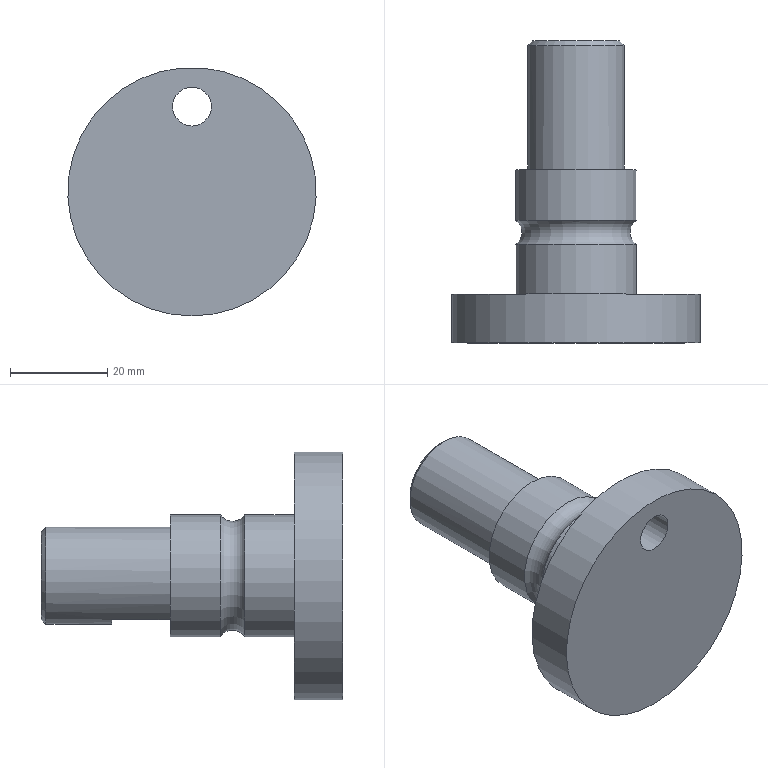Component | NX | 3_CONN_SHAFT | 1 solid | 13 faces | box 51 x 62 x 51 mm | volume 40313 mm3 | plane 6 | cylinder 5 | torus 1 | cone 1 | commonest cylinder face diameters 25 x2 51 x1 8 x1 20 x1
STEP:
#1=CARTESIAN_POINT('',(0.,0.,0.));
#2=DIRECTION('',(0.,0.,1.));
#3=DIRECTION('',(1.,0.,0.));
#4=AXIS2_PLACEMENT_3D('',#1,#2,#3);
#5=CARTESIAN_POINT('',(2.02,26.63,-37.328));
#6=VERTEX_POINT('',#5);
#7=CARTESIAN_POINT('',(2.02,26.63,-24.828));
#8=DIRECTION('',(0.,1.,0.));
#9=DIRECTION('',(0.,0.,-1.));
#10=AXIS2_PLACEMENT_3D('',#7,#8,#9);
#11=CIRCLE('',#10,12.5);
#12=CARTESIAN_POINT('',(2.02,26.63,-24.828));
#13=DIRECTION('',(0.,1.,0.));
#14=DIRECTION('',(0.,0.,-1.));
#15=AXIS2_PLACEMENT_3D('',#12,#13,#14);
#16=CYLINDRICAL_SURFACE('',#15,12.5);
#17=CARTESIAN_POINT('',(0.,0.));
#18=DIRECTION('',(1.,0.));
#19=VECTOR('',#18,1.);
#20=LINE('',#17,#19);
#21=(GEOMETRIC_REPRESENTATION_CONTEXT(2)PARAMETRIC_REPRESENTATION_CONTEXT()REPRESENTATION_CONTEXT('',''));
#22=DEFINITIONAL_REPRESENTATION('',(#20),#21);
#23=PCURVE('',#16,#22);
#24=CARTESIAN_POINT('',(2.02,26.63,-24.828));
#25=DIRECTION('',(0.,1.,0.));
#26=DIRECTION('',(0.,0.,-1.));
#27=AXIS2_PLACEMENT_3D('',#24,#25,#26);
#28=PLANE('',#27);
#29=CARTESIAN_POINT('',(0.,0.));
#30=DIRECTION('',(1.,0.));
#31=AXIS2_PLACEMENT_2D('',#29,#30);
#32=CIRCLE('',#31,12.5);
#33=(GEOMETRIC_REPRESENTATION_CONTEXT(2)PARAMETRIC_REPRESENTATION_CONTEXT()REPRESENTATION_CONTEXT('',''));
#34=DEFINITIONAL_REPRESENTATION('',(#32),#33);
#35=PCURVE('',#28,#34);
#36=SURFACE_CURVE('',#11,(#23,#35),.PCURVE_S1.);
#37=EDGE_CURVE('',#6,#6,#36,.T.);
#38=ORIENTED_EDGE('',*,*,#37,.T.);
#39=CARTESIAN_POINT('',(2.02,36.83,-37.328));
#40=VERTEX_POINT('',#39);
#41=CARTESIAN_POINT('',(2.02,26.63,-37.328));
#42=CARTESIAN_POINT('',(2.02,36.83,-37.328));
#43=B_SPLINE_CURVE_WITH_KNOTS('',1,(#41,#42),.UNSPECIFIED.,.F.,.F.,(2,2),(0.,10.2),.PIECEWISE_BEZIER_KNOTS.);
#44=CARTESIAN_POINT('',(6.283,0.));
#45=DIRECTION('',(0.,1.));
#46=VECTOR('',#45,1.);
#47=LINE('',#44,#46);
#48=(GEOMETRIC_REPRESENTATION_CONTEXT(2)PARAMETRIC_REPRESENTATION_CONTEXT()REPRESENTATION_CONTEXT('',''));
#49=DEFINITIONAL_REPRESENTATION('',(#47),#48);
#50=PCURVE('',#16,#49);
#51=CARTESIAN_POINT('',(0.,0.));
#52=DIRECTION('',(0.,1.));
#53=VECTOR('',#52,1.);
#54=LINE('',#51,#53);
#55=(GEOMETRIC_REPRESENTATION_CONTEXT(2)PARAMETRIC_REPRESENTATION_CONTEXT()REPRESENTATION_CONTEXT('',''));
#56=DEFINITIONAL_REPRESENTATION('',(#54),#55);
#57=PCURVE('',#16,#56);
#58=SEAM_CURVE('',#43,(#50,#57),.PCURVE_S1.);
#59=EDGE_CURVE('',#6,#40,#58,.T.);
#60=ORIENTED_EDGE('',*,*,#59,.T.);
#61=CARTESIAN_POINT('',(2.02,36.83,-12.328));
#62=VERTEX_POINT('',#61);
#63=CARTESIAN_POINT('',(2.02,36.83,-24.828));
#64=DIRECTION('',(0.,-1.,0.));
#65=DIRECTION('',(0.,0.,1.));
#66=AXIS2_PLACEMENT_3D('',#63,#64,#65);
#67=CIRCLE('',#66,12.5);
#68=CARTESIAN_POINT('',(9.425,10.2));
#69=DIRECTION('',(-1.,0.));
#70=VECTOR('',#69,1.);
#71=LINE('',#68,#70);
#72=(GEOMETRIC_REPRESENTATION_CONTEXT(2)PARAMETRIC_REPRESENTATION_CONTEXT()REPRESENTATION_CONTEXT('',''));
#73=DEFINITIONAL_REPRESENTATION('',(#71),#72);
#74=PCURVE('',#16,#73);
#75=CARTESIAN_POINT('',(2.02,39.33,-24.828));
#76=DIRECTION('',(0.,-1.,0.));
#77=DIRECTION('',(0.,0.,1.));
#78=AXIS2_PLACEMENT_3D('',#75,#76,#77);
#79=TOROIDAL_SURFACE('',#78,14.158,3.);
#80=CARTESIAN_POINT('',(0.,2.156));
#81=DIRECTION('',(1.,0.));
#82=VECTOR('',#81,1.);
#83=LINE('',#80,#82);
#84=(GEOMETRIC_REPRESENTATION_CONTEXT(2)PARAMETRIC_REPRESENTATION_CONTEXT()REPRESENTATION_CONTEXT('',''));
#85=DEFINITIONAL_REPRESENTATION('',(#83),#84);
#86=PCURVE('',#79,#85);
#87=SURFACE_CURVE('',#67,(#74,#86),.PCURVE_S1.);
#88=EDGE_CURVE('',#40,#62,#87,.T.);
#89=ORIENTED_EDGE('',*,*,#88,.T.);
#90=CARTESIAN_POINT('',(2.02,36.83,-24.828));
#91=DIRECTION('',(0.,-1.,0.));
#92=DIRECTION('',(0.,0.,1.));
#93=AXIS2_PLACEMENT_3D('',#90,#91,#92);
#94=CIRCLE('',#93,12.5);
#95=CARTESIAN_POINT('',(3.142,10.2));
#96=DIRECTION('',(-1.,0.));
#97=VECTOR('',#96,1.);
#98=LINE('',#95,#97);
#99=(GEOMETRIC_REPRESENTATION_CONTEXT(2)PARAMETRIC_REPRESENTATION_CONTEXT()REPRESENTATION_CONTEXT('',''));
#100=DEFINITIONAL_REPRESENTATION('',(#98),#99);
#101=PCURVE('',#16,#100);
#102=CARTESIAN_POINT('',(0.,2.156));
#103=DIRECTION('',(1.,-0.));
#104=VECTOR('',#103,1.);
#105=LINE('',#102,#104);
#106=(GEOMETRIC_REPRESENTATION_CONTEXT(2)PARAMETRIC_REPRESENTATION_CONTEXT()REPRESENTATION_CONTEXT('',''));
#107=DEFINITIONAL_REPRESENTATION('',(#105),#106);
#108=PCURVE('',#79,#107);
#109=SURFACE_CURVE('',#94,(#101,#108),.PCURVE_S1.);
#110=EDGE_CURVE('',#62,#40,#109,.T.);
#111=ORIENTED_EDGE('',*,*,#110,.T.);
#112=ORIENTED_EDGE('',*,*,#59,.F.);
#113=EDGE_LOOP('',(#38,#60,#89,#111,#112));
#114=FACE_BOUND('',#113,.T.);
#115=ADVANCED_FACE('',(#114),#16,.T.);
#116=CARTESIAN_POINT('',(2.02,26.63,-11.328));
#117=VERTEX_POINT('',#116);
#118=CARTESIAN_POINT('',(2.02,26.63,-7.328));
#119=DIRECTION('',(0.,1.,0.));
#120=DIRECTION('',(0.,0.,-1.));
#121=AXIS2_PLACEMENT_3D('',#118,#119,#120);
#122=CIRCLE('',#121,4.);
#123=CARTESIAN_POINT('',(-17.5,0.));
#124=DIRECTION('',(1.,0.));
#125=AXIS2_PLACEMENT_2D('',#123,#124);
#126=CIRCLE('',#125,4.);
#127=(GEOMETRIC_REPRESENTATION_CONTEXT(2)PARAMETRIC_REPRESENTATION_CONTEXT()REPRESENTATION_CONTEXT('',''));
#128=DEFINITIONAL_REPRESENTATION('',(#126),#127);
#129=PCURVE('',#28,#128);
#130=CARTESIAN_POINT('',(2.02,33.63,-7.328));
#131=DIRECTION('',(0.,-1.,0.));
#132=DIRECTION('',(0.,0.,1.));
#133=AXIS2_PLACEMENT_3D('',#130,#131,#132);
#134=CYLINDRICAL_SURFACE('',#133,4.);
#135=CARTESIAN_POINT('',(9.425,7.));
#136=DIRECTION('',(-1.,0.));
#137=VECTOR('',#136,1.);
#138=LINE('',#135,#137);
#139=(GEOMETRIC_REPRESENTATION_CONTEXT(2)PARAMETRIC_REPRESENTATION_CONTEXT()REPRESENTATION_CONTEXT('',''));
#140=DEFINITIONAL_REPRESENTATION('',(#138),#139);
#141=PCURVE('',#134,#140);
#142=SURFACE_CURVE('',#122,(#129,#141),.PCURVE_S1.);
#143=EDGE_CURVE('',#117,#117,#142,.T.);
#144=ORIENTED_EDGE('',*,*,#143,.F.);
#145=EDGE_LOOP('',(#144));
#146=FACE_BOUND('',#145,.T.);
#147=ORIENTED_EDGE('',*,*,#37,.F.);
#148=EDGE_LOOP('',(#147));
#149=FACE_BOUND('',#148,.T.);
#150=CARTESIAN_POINT('',(2.02,26.63,-50.328));
#151=VERTEX_POINT('',#150);
#152=CARTESIAN_POINT('',(2.02,26.63,-24.828));
#153=DIRECTION('',(0.,-1.,0.));
#154=DIRECTION('',(0.,0.,-1.));
#155=AXIS2_PLACEMENT_3D('',#152,#153,#154);
#156=CIRCLE('',#155,25.5);
#157=CARTESIAN_POINT('',(25.5,0.));
#158=CARTESIAN_POINT('',(25.5,-44.167));
#159=CARTESIAN_POINT('',(-12.75,-22.084));
#160=CARTESIAN_POINT('',(-51.,-0.));
#161=CARTESIAN_POINT('',(-12.75,22.084));
#162=CARTESIAN_POINT('',(25.5,44.167));
#163=CARTESIAN_POINT('',(25.5,0.));
#164=(BOUNDED_CURVE()B_SPLINE_CURVE(2,(#157,#158,#159,#160,#161,#162,#163),.UNSPECIFIED.,.T.,.F.)B_SPLINE_CURVE_WITH_KNOTS((1,2,2,2,2,1),(-2.094,0.,2.094,4.189,6.283,8.378),.UNSPECIFIED.)CURVE()GEOMETRIC_REPRESENTATION_ITEM()RATIONAL_B_SPLINE_CURVE((1.,0.5,1.,0.5,1.,0.5,1.))REPRESENTATION_ITEM(''));
#165=(GEOMETRIC_REPRESENTATION_CONTEXT(2)PARAMETRIC_REPRESENTATION_CONTEXT()REPRESENTATION_CONTEXT('',''));
#166=DEFINITIONAL_REPRESENTATION('',(#164),#165);
#167=PCURVE('',#28,#166);
#168=CARTESIAN_POINT('',(2.02,16.63,-24.828));
#169=DIRECTION('',(0.,1.,0.));
#170=DIRECTION('',(0.,0.,-1.));
#171=AXIS2_PLACEMENT_3D('',#168,#169,#170);
#172=CYLINDRICAL_SURFACE('',#171,25.5);
#173=CARTESIAN_POINT('',(6.283,10.));
#174=DIRECTION('',(-1.,0.));
#175=VECTOR('',#174,1.);
#176=LINE('',#173,#175);
#177=(GEOMETRIC_REPRESENTATION_CONTEXT(2)PARAMETRIC_REPRESENTATION_CONTEXT()REPRESENTATION_CONTEXT('',''));
#178=DEFINITIONAL_REPRESENTATION('',(#176),#177);
#179=PCURVE('',#172,#178);
#180=SURFACE_CURVE('',#156,(#167,#179),.PCURVE_S1.);
#181=EDGE_CURVE('',#151,#151,#180,.T.);
#182=ORIENTED_EDGE('',*,*,#181,.F.);
#183=EDGE_LOOP('',(#182));
#184=FACE_BOUND('',#183,.T.);
#185=ADVANCED_FACE('',(#146,#149,#184),#28,.T.);
#186=CARTESIAN_POINT('',(2.02,16.63,-11.328));
#187=VERTEX_POINT('',#186);
#188=CARTESIAN_POINT('',(2.02,16.63,-7.328));
#189=DIRECTION('',(0.,-1.,0.));
#190=DIRECTION('',(-0.,0.,-1.));
#191=AXIS2_PLACEMENT_3D('',#188,#189,#190);
#192=CIRCLE('',#191,4.);
#193=CARTESIAN_POINT('',(2.02,16.63,-24.828));
#194=DIRECTION('',(0.,-1.,0.));
#195=DIRECTION('',(0.,0.,1.));
#196=AXIS2_PLACEMENT_3D('',#193,#194,#195);
#197=PLANE('',#196);
#198=CARTESIAN_POINT('',(17.5,0.));
#199=DIRECTION('',(-1.,0.));
#200=AXIS2_PLACEMENT_2D('',#198,#199);
#201=CIRCLE('',#200,4.);
#202=(GEOMETRIC_REPRESENTATION_CONTEXT(2)PARAMETRIC_REPRESENTATION_CONTEXT()REPRESENTATION_CONTEXT('',''));
#203=DEFINITIONAL_REPRESENTATION('',(#201),#202);
#204=PCURVE('',#197,#203);
#205=CARTESIAN_POINT('',(3.142,17.));
#206=DIRECTION('',(1.,0.));
#207=VECTOR('',#206,1.);
#208=LINE('',#205,#207);
#209=(GEOMETRIC_REPRESENTATION_CONTEXT(2)PARAMETRIC_REPRESENTATION_CONTEXT()REPRESENTATION_CONTEXT('',''));
#210=DEFINITIONAL_REPRESENTATION('',(#208),#209);
#211=PCURVE('',#134,#210);
#212=SURFACE_CURVE('',#192,(#204,#211),.PCURVE_S1.);
#213=EDGE_CURVE('',#187,#187,#212,.T.);
#214=ORIENTED_EDGE('',*,*,#213,.F.);
#215=EDGE_LOOP('',(#214));
#216=FACE_BOUND('',#215,.T.);
#217=CARTESIAN_POINT('',(2.02,16.63,-50.328));
#218=VERTEX_POINT('',#217);
#219=CARTESIAN_POINT('',(2.02,16.63,-24.828));
#220=DIRECTION('',(0.,1.,0.));
#221=DIRECTION('',(0.,0.,-1.));
#222=AXIS2_PLACEMENT_3D('',#219,#220,#221);
#223=CIRCLE('',#222,25.5);
#224=CARTESIAN_POINT('',(-25.5,0.));
#225=CARTESIAN_POINT('',(-25.5,44.167));
#226=CARTESIAN_POINT('',(12.75,22.084));
#227=CARTESIAN_POINT('',(51.,0.));
#228=CARTESIAN_POINT('',(12.75,-22.084));
#229=CARTESIAN_POINT('',(-25.5,-44.167));
#230=CARTESIAN_POINT('',(-25.5,0.));
#231=(BOUNDED_CURVE()B_SPLINE_CURVE(2,(#224,#225,#226,#227,#228,#229,#230),.UNSPECIFIED.,.T.,.F.)B_SPLINE_CURVE_WITH_KNOTS((1,2,2,2,2,1),(-2.094,0.,2.094,4.189,6.283,8.378),.UNSPECIFIED.)CURVE()GEOMETRIC_REPRESENTATION_ITEM()RATIONAL_B_SPLINE_CURVE((1.,0.5,1.,0.5,1.,0.5,1.))REPRESENTATION_ITEM(''));
#232=(GEOMETRIC_REPRESENTATION_CONTEXT(2)PARAMETRIC_REPRESENTATION_CONTEXT()REPRESENTATION_CONTEXT('',''));
#233=DEFINITIONAL_REPRESENTATION('',(#231),#232);
#234=PCURVE('',#197,#233);
#235=CARTESIAN_POINT('',(0.,0.));
#236=DIRECTION('',(1.,0.));
#237=VECTOR('',#236,1.);
#238=LINE('',#235,#237);
#239=(GEOMETRIC_REPRESENTATION_CONTEXT(2)PARAMETRIC_REPRESENTATION_CONTEXT()REPRESENTATION_CONTEXT('',''));
#240=DEFINITIONAL_REPRESENTATION('',(#238),#239);
#241=PCURVE('',#172,#240);
#242=SURFACE_CURVE('',#223,(#234,#241),.PCURVE_S1.);
#243=EDGE_CURVE('',#218,#218,#242,.T.);
#244=ORIENTED_EDGE('',*,*,#243,.F.);
#245=EDGE_LOOP('',(#244));
#246=FACE_BOUND('',#245,.T.);
#247=ADVANCED_FACE('',(#216,#246),#197,.T.);
#248=ORIENTED_EDGE('',*,*,#181,.T.);
#249=CARTESIAN_POINT('',(2.02,16.63,-50.328));
#250=CARTESIAN_POINT('',(2.02,26.63,-50.328));
#251=B_SPLINE_CURVE_WITH_KNOTS('',1,(#249,#250),.UNSPECIFIED.,.F.,.F.,(2,2),(0.,10.),.PIECEWISE_BEZIER_KNOTS.);
#252=CARTESIAN_POINT('',(0.,0.));
#253=DIRECTION('',(0.,1.));
#254=VECTOR('',#253,1.);
#255=LINE('',#252,#254);
#256=(GEOMETRIC_REPRESENTATION_CONTEXT(2)PARAMETRIC_REPRESENTATION_CONTEXT()REPRESENTATION_CONTEXT('',''));
#257=DEFINITIONAL_REPRESENTATION('',(#255),#256);
#258=PCURVE('',#172,#257);
#259=CARTESIAN_POINT('',(6.283,0.));
#260=DIRECTION('',(0.,1.));
#261=VECTOR('',#260,1.);
#262=LINE('',#259,#261);
#263=(GEOMETRIC_REPRESENTATION_CONTEXT(2)PARAMETRIC_REPRESENTATION_CONTEXT()REPRESENTATION_CONTEXT('',''));
#264=DEFINITIONAL_REPRESENTATION('',(#262),#263);
#265=PCURVE('',#172,#264);
#266=SEAM_CURVE('',#251,(#258,#265),.PCURVE_S1.);
#267=EDGE_CURVE('',#218,#151,#266,.T.);
#268=ORIENTED_EDGE('',*,*,#267,.F.);
#269=ORIENTED_EDGE('',*,*,#243,.T.);
#270=ORIENTED_EDGE('',*,*,#267,.T.);
#271=EDGE_LOOP('',(#248,#268,#269,#270));
#272=FACE_BOUND('',#271,.T.);
#273=ADVANCED_FACE('',(#272),#172,.T.);
#274=ORIENTED_EDGE('',*,*,#143,.F.);
#275=CARTESIAN_POINT('',(2.02,26.63,-11.328));
#276=CARTESIAN_POINT('',(2.02,16.63,-11.328));
#277=B_SPLINE_CURVE_WITH_KNOTS('',1,(#275,#276),.UNSPECIFIED.,.F.,.F.,(2,2),(7.,17.),.PIECEWISE_BEZIER_KNOTS.);
#278=CARTESIAN_POINT('',(9.425,0.));
#279=DIRECTION('',(0.,1.));
#280=VECTOR('',#279,1.);
#281=LINE('',#278,#280);
#282=(GEOMETRIC_REPRESENTATION_CONTEXT(2)PARAMETRIC_REPRESENTATION_CONTEXT()REPRESENTATION_CONTEXT('',''));
#283=DEFINITIONAL_REPRESENTATION('',(#281),#282);
#284=PCURVE('',#134,#283);
#285=CARTESIAN_POINT('',(3.142,0.));
#286=DIRECTION('',(0.,1.));
#287=VECTOR('',#286,1.);
#288=LINE('',#285,#287);
#289=(GEOMETRIC_REPRESENTATION_CONTEXT(2)PARAMETRIC_REPRESENTATION_CONTEXT()REPRESENTATION_CONTEXT('',''));
#290=DEFINITIONAL_REPRESENTATION('',(#288),#289);
#291=PCURVE('',#134,#290);
#292=SEAM_CURVE('',#277,(#284,#291),.PCURVE_S1.);
#293=EDGE_CURVE('',#117,#187,#292,.T.);
#294=ORIENTED_EDGE('',*,*,#293,.T.);
#295=ORIENTED_EDGE('',*,*,#213,.F.);
#296=ORIENTED_EDGE('',*,*,#293,.F.);
#297=EDGE_LOOP('',(#274,#294,#295,#296));
#298=FACE_BOUND('',#297,.F.);
#299=ADVANCED_FACE('',(#298),#134,.F.);
#300=CARTESIAN_POINT('',(2.02,41.83,-12.328));
#301=VERTEX_POINT('',#300);
#302=CARTESIAN_POINT('',(2.02,41.83,-37.328));
#303=VERTEX_POINT('',#302);
#304=CARTESIAN_POINT('',(2.02,41.83,-24.828));
#305=DIRECTION('',(0.,1.,0.));
#306=DIRECTION('',(0.,0.,1.));
#307=AXIS2_PLACEMENT_3D('',#304,#305,#306);
#308=CIRCLE('',#307,12.5);
#309=CARTESIAN_POINT('',(6.283,4.127));
#310=DIRECTION('',(-1.,0.));
#311=VECTOR('',#310,1.);
#312=LINE('',#309,#311);
#313=(GEOMETRIC_REPRESENTATION_CONTEXT(2)PARAMETRIC_REPRESENTATION_CONTEXT()REPRESENTATION_CONTEXT('',''));
#314=DEFINITIONAL_REPRESENTATION('',(#312),#313);
#315=PCURVE('',#79,#314);
#316=CARTESIAN_POINT('',(2.02,26.63,-24.828));
#317=DIRECTION('',(0.,1.,0.));
#318=DIRECTION('',(0.,0.,-1.));
#319=AXIS2_PLACEMENT_3D('',#316,#317,#318);
#320=CYLINDRICAL_SURFACE('',#319,12.5);
#321=CARTESIAN_POINT('',(3.142,15.2));
#322=DIRECTION('',(1.,0.));
#323=VECTOR('',#322,1.);
#324=LINE('',#321,#323);
#325=(GEOMETRIC_REPRESENTATION_CONTEXT(2)PARAMETRIC_REPRESENTATION_CONTEXT()REPRESENTATION_CONTEXT('',''));
#326=DEFINITIONAL_REPRESENTATION('',(#324),#325);
#327=PCURVE('',#320,#326);
#328=SURFACE_CURVE('',#308,(#315,#327),.PCURVE_S1.);
#329=EDGE_CURVE('',#301,#303,#328,.T.);
#330=ORIENTED_EDGE('',*,*,#329,.T.);
#331=CARTESIAN_POINT('',(2.02,41.83,-24.828));
#332=DIRECTION('',(0.,1.,0.));
#333=DIRECTION('',(0.,0.,1.));
#334=AXIS2_PLACEMENT_3D('',#331,#332,#333);
#335=CIRCLE('',#334,12.5);
#336=CARTESIAN_POINT('',(6.283,4.127));
#337=DIRECTION('',(-1.,0.));
#338=VECTOR('',#337,1.);
#339=LINE('',#336,#338);
#340=(GEOMETRIC_REPRESENTATION_CONTEXT(2)PARAMETRIC_REPRESENTATION_CONTEXT()REPRESENTATION_CONTEXT('',''));
#341=DEFINITIONAL_REPRESENTATION('',(#339),#340);
#342=PCURVE('',#79,#341);
#343=CARTESIAN_POINT('',(-3.142,15.2));
#344=DIRECTION('',(1.,0.));
#345=VECTOR('',#344,1.);
#346=LINE('',#343,#345);
#347=(GEOMETRIC_REPRESENTATION_CONTEXT(2)PARAMETRIC_REPRESENTATION_CONTEXT()REPRESENTATION_CONTEXT('',''));
#348=DEFINITIONAL_REPRESENTATION('',(#346),#347);
#349=PCURVE('',#320,#348);
#350=SURFACE_CURVE('',#335,(#342,#349),.PCURVE_S1.);
#351=EDGE_CURVE('',#303,#301,#350,.T.);
#352=ORIENTED_EDGE('',*,*,#351,.T.);
#353=CARTESIAN_POINT('',(2.02,36.83,-12.328));
#354=CARTESIAN_POINT('',(2.02,37.393,-13.177));
#355=CARTESIAN_POINT('',(2.02,38.273,-13.763));
#356=CARTESIAN_POINT('',(2.02,39.33,-13.974));
#357=CARTESIAN_POINT('',(2.02,40.388,-13.763));
#358=CARTESIAN_POINT('',(2.02,41.267,-13.177));
#359=CARTESIAN_POINT('',(2.02,41.83,-12.328));
#360=(BOUNDED_CURVE()B_SPLINE_CURVE(6,(#353,#354,#355,#356,#357,#358,#359),.UNSPECIFIED.,.F.,.F.)B_SPLINE_CURVE_WITH_KNOTS((7,7),(2.156,4.127),.PIECEWISE_BEZIER_KNOTS.)CURVE()GEOMETRIC_REPRESENTATION_ITEM()RATIONAL_B_SPLINE_CURVE((1.05,1.016,0.9967,0.9906,0.9967,1.016,1.05))REPRESENTATION_ITEM(''));
#361=CARTESIAN_POINT('',(0.,0.));
#362=DIRECTION('',(0.,1.));
#363=VECTOR('',#362,1.);
#364=LINE('',#361,#363);
#365=(GEOMETRIC_REPRESENTATION_CONTEXT(2)PARAMETRIC_REPRESENTATION_CONTEXT()REPRESENTATION_CONTEXT('',''));
#366=DEFINITIONAL_REPRESENTATION('',(#364),#365);
#367=PCURVE('',#79,#366);
#368=CARTESIAN_POINT('',(6.283,0.));
#369=DIRECTION('',(0.,1.));
#370=VECTOR('',#369,1.);
#371=LINE('',#368,#370);
#372=(GEOMETRIC_REPRESENTATION_CONTEXT(2)PARAMETRIC_REPRESENTATION_CONTEXT()REPRESENTATION_CONTEXT('',''));
#373=DEFINITIONAL_REPRESENTATION('',(#371),#372);
#374=PCURVE('',#79,#373);
#375=SEAM_CURVE('',#360,(#367,#374),.PCURVE_S1.);
#376=EDGE_CURVE('',#62,#301,#375,.T.);
#377=ORIENTED_EDGE('',*,*,#376,.F.);
#378=ORIENTED_EDGE('',*,*,#110,.T.);
#379=ORIENTED_EDGE('',*,*,#88,.T.);
#380=ORIENTED_EDGE('',*,*,#376,.T.);
#381=EDGE_LOOP('',(#330,#352,#377,#378,#379,#380));
#382=FACE_BOUND('',#381,.F.);
#383=ADVANCED_FACE('',(#382),#79,.F.);
#384=CARTESIAN_POINT('',(2.02,78.63,-33.828));
#385=VERTEX_POINT('',#384);
#386=CARTESIAN_POINT('',(2.02,78.63,-24.828));
#387=DIRECTION('',(0.,1.,0.));
#388=DIRECTION('',(0.,0.,-1.));
#389=AXIS2_PLACEMENT_3D('',#386,#387,#388);
#390=CIRCLE('',#389,9.);
#391=CARTESIAN_POINT('',(2.02,78.63,-24.828));
#392=DIRECTION('',(0.,1.,0.));
#393=DIRECTION('',(0.,0.,-1.));
#394=AXIS2_PLACEMENT_3D('',#391,#392,#393);
#395=PLANE('',#394);
#396=CARTESIAN_POINT('',(0.,0.));
#397=DIRECTION('',(1.,0.));
#398=AXIS2_PLACEMENT_2D('',#396,#397);
#399=CIRCLE('',#398,9.);
#400=(GEOMETRIC_REPRESENTATION_CONTEXT(2)PARAMETRIC_REPRESENTATION_CONTEXT()REPRESENTATION_CONTEXT('',''));
#401=DEFINITIONAL_REPRESENTATION('',(#399),#400);
#402=PCURVE('',#395,#401);
#403=CARTESIAN_POINT('',(2.02,77.63,-24.828));
#404=DIRECTION('',(0.,-1.,0.));
#405=DIRECTION('',(0.,0.,1.));
#406=AXIS2_PLACEMENT_3D('',#403,#404,#405);
#407=CONICAL_SURFACE('',#406,10.,0.7854);
#408=CARTESIAN_POINT('',(9.425,-1.));
#409=DIRECTION('',(-1.,0.));
#410=VECTOR('',#409,1.);
#411=LINE('',#408,#410);
#412=(GEOMETRIC_REPRESENTATION_CONTEXT(2)PARAMETRIC_REPRESENTATION_CONTEXT()REPRESENTATION_CONTEXT('',''));
#413=DEFINITIONAL_REPRESENTATION('',(#411),#412);
#414=PCURVE('',#407,#413);
#415=SURFACE_CURVE('',#390,(#402,#414),.PCURVE_S1.);
#416=EDGE_CURVE('',#385,#385,#415,.T.);
#417=ORIENTED_EDGE('',*,*,#416,.T.);
#418=EDGE_LOOP('',(#417));
#419=FACE_BOUND('',#418,.T.);
#420=ADVANCED_FACE('',(#419),#395,.T.);
#421=CARTESIAN_POINT('',(6.379,64.13,-33.828));
#422=VERTEX_POINT('',#421);
#423=CARTESIAN_POINT('',(2.02,64.13,-34.828));
#424=VERTEX_POINT('',#423);
#425=CARTESIAN_POINT('',(2.02,64.13,-24.828));
#426=DIRECTION('',(0.,1.,0.));
#427=DIRECTION('',(0.,0.,-1.));
#428=AXIS2_PLACEMENT_3D('',#425,#426,#427);
#429=CIRCLE('',#428,10.);
#430=CARTESIAN_POINT('',(2.02,64.13,-24.828));
#431=DIRECTION('',(0.,-1.,0.));
#432=DIRECTION('',(0.,0.,1.));
#433=AXIS2_PLACEMENT_3D('',#430,#431,#432);
#434=PLANE('',#433);
#435=CARTESIAN_POINT('',(-10.,0.));
#436=CARTESIAN_POINT('',(-10.,17.321));
#437=CARTESIAN_POINT('',(5.,8.66));
#438=CARTESIAN_POINT('',(20.,0.));
#439=CARTESIAN_POINT('',(5.,-8.66));
#440=CARTESIAN_POINT('',(-10.,-17.321));
#441=CARTESIAN_POINT('',(-10.,0.));
#442=(BOUNDED_CURVE()B_SPLINE_CURVE(2,(#435,#436,#437,#438,#439,#440,#441),.UNSPECIFIED.,.T.,.F.)B_SPLINE_CURVE_WITH_KNOTS((1,2,2,2,2,1),(-2.094,0.,2.094,4.189,6.283,8.378),.UNSPECIFIED.)CURVE()GEOMETRIC_REPRESENTATION_ITEM()RATIONAL_B_SPLINE_CURVE((1.,0.5,1.,0.5,1.,0.5,1.))REPRESENTATION_ITEM(''));
#443=(GEOMETRIC_REPRESENTATION_CONTEXT(2)PARAMETRIC_REPRESENTATION_CONTEXT()REPRESENTATION_CONTEXT('',''));
#444=DEFINITIONAL_REPRESENTATION('',(#442),#443);
#445=PCURVE('',#434,#444);
#446=CARTESIAN_POINT('',(2.02,52.13,-24.828));
#447=DIRECTION('',(0.,1.,0.));
#448=DIRECTION('',(0.,0.,-1.));
#449=AXIS2_PLACEMENT_3D('',#446,#447,#448);
#450=CYLINDRICAL_SURFACE('',#449,10.);
#451=CARTESIAN_POINT('',(0.,12.));
#452=DIRECTION('',(1.,0.));
#453=VECTOR('',#452,1.);
#454=LINE('',#451,#453);
#455=(GEOMETRIC_REPRESENTATION_CONTEXT(2)PARAMETRIC_REPRESENTATION_CONTEXT()REPRESENTATION_CONTEXT('',''));
#456=DEFINITIONAL_REPRESENTATION('',(#454),#455);
#457=PCURVE('',#450,#456);
#458=SURFACE_CURVE('',#429,(#445,#457),.PCURVE_S1.);
#459=EDGE_CURVE('',#422,#424,#458,.T.);
#460=ORIENTED_EDGE('',*,*,#459,.F.);
#461=CARTESIAN_POINT('',(-2.339,64.13,-33.828));
#462=VERTEX_POINT('',#461);
#463=CARTESIAN_POINT('',(2.02,64.13,-33.828));
#464=DIRECTION('',(-1.,0.,0.));
#465=VECTOR('',#464,1.);
#466=LINE('',#463,#465);
#467=CARTESIAN_POINT('',(-9.,0.));
#468=DIRECTION('',(0.,1.));
#469=VECTOR('',#468,1.);
#470=LINE('',#467,#469);
#471=(GEOMETRIC_REPRESENTATION_CONTEXT(2)PARAMETRIC_REPRESENTATION_CONTEXT()REPRESENTATION_CONTEXT('',''));
#472=DEFINITIONAL_REPRESENTATION('',(#470),#471);
#473=PCURVE('',#434,#472);
#474=CARTESIAN_POINT('',(2.02,16.63,-33.828));
#475=DIRECTION('',(0.,0.,-1.));
#476=DIRECTION('',(0.,-1.,0.));
#477=AXIS2_PLACEMENT_3D('',#474,#475,#476);
#478=PLANE('',#477);
#479=CARTESIAN_POINT('',(-47.5,0.));
#480=DIRECTION('',(0.,1.));
#481=VECTOR('',#480,1.);
#482=LINE('',#479,#481);
#483=(GEOMETRIC_REPRESENTATION_CONTEXT(2)PARAMETRIC_REPRESENTATION_CONTEXT()REPRESENTATION_CONTEXT('',''));
#484=DEFINITIONAL_REPRESENTATION('',(#482),#483);
#485=PCURVE('',#478,#484);
#486=SURFACE_CURVE('',#466,(#473,#485),.PCURVE_S1.);
#487=EDGE_CURVE('',#422,#462,#486,.T.);
#488=ORIENTED_EDGE('',*,*,#487,.T.);
#489=CARTESIAN_POINT('',(2.02,64.13,-24.828));
#490=DIRECTION('',(0.,1.,0.));
#491=DIRECTION('',(0.,0.,-1.));
#492=AXIS2_PLACEMENT_3D('',#489,#490,#491);
#493=CIRCLE('',#492,10.);
#494=CARTESIAN_POINT('',(-10.,0.));
#495=CARTESIAN_POINT('',(-10.,17.321));
#496=CARTESIAN_POINT('',(5.,8.66));
#497=CARTESIAN_POINT('',(20.,0.));
#498=CARTESIAN_POINT('',(5.,-8.66));
#499=CARTESIAN_POINT('',(-10.,-17.321));
#500=CARTESIAN_POINT('',(-10.,0.));
#501=(BOUNDED_CURVE()B_SPLINE_CURVE(2,(#494,#495,#496,#497,#498,#499,#500),.UNSPECIFIED.,.T.,.F.)B_SPLINE_CURVE_WITH_KNOTS((1,2,2,2,2,1),(-2.094,0.,2.094,4.189,6.283,8.378),.UNSPECIFIED.)CURVE()GEOMETRIC_REPRESENTATION_ITEM()RATIONAL_B_SPLINE_CURVE((1.,0.5,1.,0.5,1.,0.5,1.))REPRESENTATION_ITEM(''));
#502=(GEOMETRIC_REPRESENTATION_CONTEXT(2)PARAMETRIC_REPRESENTATION_CONTEXT()REPRESENTATION_CONTEXT('',''));
#503=DEFINITIONAL_REPRESENTATION('',(#501),#502);
#504=PCURVE('',#434,#503);
#505=CARTESIAN_POINT('',(-6.283,12.));
#506=DIRECTION('',(1.,0.));
#507=VECTOR('',#506,1.);
#508=LINE('',#505,#507);
#509=(GEOMETRIC_REPRESENTATION_CONTEXT(2)PARAMETRIC_REPRESENTATION_CONTEXT()REPRESENTATION_CONTEXT('',''));
#510=DEFINITIONAL_REPRESENTATION('',(#508),#509);
#511=PCURVE('',#450,#510);
#512=SURFACE_CURVE('',#493,(#504,#511),.PCURVE_S1.);
#513=EDGE_CURVE('',#424,#462,#512,.T.);
#514=ORIENTED_EDGE('',*,*,#513,.F.);
#515=EDGE_LOOP('',(#460,#488,#514));
#516=FACE_BOUND('',#515,.T.);
#517=ADVANCED_FACE('',(#516),#434,.T.);
#518=CARTESIAN_POINT('',(-2.339,52.13,-33.828));
#519=VERTEX_POINT('',#518);
#520=CARTESIAN_POINT('',(-2.339,52.13,-33.828));
#521=DIRECTION('',(0.,-1.,0.));
#522=VECTOR('',#521,1.);
#523=LINE('',#520,#522);
#524=CARTESIAN_POINT('',(-35.5,4.359));
#525=DIRECTION('',(1.,0.));
#526=VECTOR('',#525,1.);
#527=LINE('',#524,#526);
#528=(GEOMETRIC_REPRESENTATION_CONTEXT(2)PARAMETRIC_REPRESENTATION_CONTEXT()REPRESENTATION_CONTEXT('',''));
#529=DEFINITIONAL_REPRESENTATION('',(#527),#528);
#530=PCURVE('',#478,#529);
#531=CARTESIAN_POINT('',(0.451,0.));
#532=DIRECTION('',(0.,-1.));
#533=VECTOR('',#532,1.);
#534=LINE('',#531,#533);
#535=(GEOMETRIC_REPRESENTATION_CONTEXT(2)PARAMETRIC_REPRESENTATION_CONTEXT()REPRESENTATION_CONTEXT('',''));
#536=DEFINITIONAL_REPRESENTATION('',(#534),#535);
#537=PCURVE('',#450,#536);
#538=SURFACE_CURVE('',#523,(#530,#537),.PCURVE_S1.);
#539=EDGE_CURVE('',#462,#519,#538,.T.);
#540=ORIENTED_EDGE('',*,*,#539,.F.);
#541=ORIENTED_EDGE('',*,*,#487,.F.);
#542=CARTESIAN_POINT('',(6.379,52.13,-33.828));
#543=VERTEX_POINT('',#542);
#544=CARTESIAN_POINT('',(6.379,52.13,-33.828));
#545=DIRECTION('',(0.,1.,0.));
#546=VECTOR('',#545,1.);
#547=LINE('',#544,#546);
#548=CARTESIAN_POINT('',(-35.5,-4.359));
#549=DIRECTION('',(-1.,0.));
#550=VECTOR('',#549,1.);
#551=LINE('',#548,#550);
#552=(GEOMETRIC_REPRESENTATION_CONTEXT(2)PARAMETRIC_REPRESENTATION_CONTEXT()REPRESENTATION_CONTEXT('',''));
#553=DEFINITIONAL_REPRESENTATION('',(#551),#552);
#554=PCURVE('',#478,#553);
#555=CARTESIAN_POINT('',(5.832,0.));
#556=DIRECTION('',(0.,1.));
#557=VECTOR('',#556,1.);
#558=LINE('',#555,#557);
#559=(GEOMETRIC_REPRESENTATION_CONTEXT(2)PARAMETRIC_REPRESENTATION_CONTEXT()REPRESENTATION_CONTEXT('',''));
#560=DEFINITIONAL_REPRESENTATION('',(#558),#559);
#561=PCURVE('',#450,#560);
#562=SURFACE_CURVE('',#547,(#554,#561),.PCURVE_S1.);
#563=EDGE_CURVE('',#543,#422,#562,.T.);
#564=ORIENTED_EDGE('',*,*,#563,.F.);
#565=CARTESIAN_POINT('',(2.02,52.13,-33.828));
#566=DIRECTION('',(1.,0.,0.));
#567=VECTOR('',#566,1.);
#568=LINE('',#565,#567);
#569=CARTESIAN_POINT('',(-35.5,0.));
#570=DIRECTION('',(0.,-1.));
#571=VECTOR('',#570,1.);
#572=LINE('',#569,#571);
#573=(GEOMETRIC_REPRESENTATION_CONTEXT(2)PARAMETRIC_REPRESENTATION_CONTEXT()REPRESENTATION_CONTEXT('',''));
#574=DEFINITIONAL_REPRESENTATION('',(#572),#573);
#575=PCURVE('',#478,#574);
#576=CARTESIAN_POINT('',(2.02,52.13,-24.828));
#577=DIRECTION('',(0.,1.,0.));
#578=DIRECTION('',(0.,0.,-1.));
#579=AXIS2_PLACEMENT_3D('',#576,#577,#578);
#580=PLANE('',#579);
#581=CARTESIAN_POINT('',(9.,0.));
#582=DIRECTION('',(0.,-1.));
#583=VECTOR('',#582,1.);
#584=LINE('',#581,#583);
#585=(GEOMETRIC_REPRESENTATION_CONTEXT(2)PARAMETRIC_REPRESENTATION_CONTEXT()REPRESENTATION_CONTEXT('',''));
#586=DEFINITIONAL_REPRESENTATION('',(#584),#585);
#587=PCURVE('',#580,#586);
#588=SURFACE_CURVE('',#568,(#575,#587),.PCURVE_S1.);
#589=EDGE_CURVE('',#519,#543,#588,.T.);
#590=ORIENTED_EDGE('',*,*,#589,.F.);
#591=EDGE_LOOP('',(#540,#541,#564,#590));
#592=FACE_BOUND('',#591,.T.);
#593=ADVANCED_FACE('',(#592),#478,.T.);
#594=CARTESIAN_POINT('',(2.02,77.63,-34.828));
#595=VERTEX_POINT('',#594);
#596=CARTESIAN_POINT('',(2.02,77.63,-24.828));
#597=DIRECTION('',(0.,-1.,0.));
#598=DIRECTION('',(0.,0.,-1.));
#599=AXIS2_PLACEMENT_3D('',#596,#597,#598);
#600=CIRCLE('',#599,10.);
#601=CARTESIAN_POINT('',(6.283,25.5));
#602=DIRECTION('',(-1.,0.));
#603=VECTOR('',#602,1.);
#604=LINE('',#601,#603);
#605=(GEOMETRIC_REPRESENTATION_CONTEXT(2)PARAMETRIC_REPRESENTATION_CONTEXT()REPRESENTATION_CONTEXT('',''));
#606=DEFINITIONAL_REPRESENTATION('',(#604),#605);
#607=PCURVE('',#450,#606);
#608=CARTESIAN_POINT('',(3.142,0.));
#609=DIRECTION('',(1.,0.));
#610=VECTOR('',#609,1.);
#611=LINE('',#608,#610);
#612=(GEOMETRIC_REPRESENTATION_CONTEXT(2)PARAMETRIC_REPRESENTATION_CONTEXT()REPRESENTATION_CONTEXT('',''));
#613=DEFINITIONAL_REPRESENTATION('',(#611),#612);
#614=PCURVE('',#407,#613);
#615=SURFACE_CURVE('',#600,(#607,#614),.PCURVE_S1.);
#616=EDGE_CURVE('',#595,#595,#615,.T.);
#617=ORIENTED_EDGE('',*,*,#616,.T.);
#618=CARTESIAN_POINT('',(2.02,64.13,-34.828));
#619=CARTESIAN_POINT('',(2.02,77.63,-34.828));
#620=B_SPLINE_CURVE_WITH_KNOTS('',1,(#618,#619),.UNSPECIFIED.,.F.,.F.,(2,2),(12.,25.5),.PIECEWISE_BEZIER_KNOTS.);
#621=CARTESIAN_POINT('',(0.,0.));
#622=DIRECTION('',(0.,1.));
#623=VECTOR('',#622,1.);
#624=LINE('',#621,#623);
#625=(GEOMETRIC_REPRESENTATION_CONTEXT(2)PARAMETRIC_REPRESENTATION_CONTEXT()REPRESENTATION_CONTEXT('',''));
#626=DEFINITIONAL_REPRESENTATION('',(#624),#625);
#627=PCURVE('',#450,#626);
#628=CARTESIAN_POINT('',(6.283,0.));
#629=DIRECTION('',(0.,1.));
#630=VECTOR('',#629,1.);
#631=LINE('',#628,#630);
#632=(GEOMETRIC_REPRESENTATION_CONTEXT(2)PARAMETRIC_REPRESENTATION_CONTEXT()REPRESENTATION_CONTEXT('',''));
#633=DEFINITIONAL_REPRESENTATION('',(#631),#632);
#634=PCURVE('',#450,#633);
#635=SEAM_CURVE('',#620,(#627,#634),.PCURVE_S1.);
#636=EDGE_CURVE('',#424,#595,#635,.T.);
#637=ORIENTED_EDGE('',*,*,#636,.F.);
#638=ORIENTED_EDGE('',*,*,#513,.T.);
#639=ORIENTED_EDGE('',*,*,#539,.T.);
#640=CARTESIAN_POINT('',(2.02,52.13,-24.828));
#641=DIRECTION('',(0.,1.,0.));
#642=DIRECTION('',(0.,0.,-1.));
#643=AXIS2_PLACEMENT_3D('',#640,#641,#642);
#644=CIRCLE('',#643,10.);
#645=CARTESIAN_POINT('',(0.,0.));
#646=DIRECTION('',(1.,0.));
#647=VECTOR('',#646,1.);
#648=LINE('',#645,#647);
#649=(GEOMETRIC_REPRESENTATION_CONTEXT(2)PARAMETRIC_REPRESENTATION_CONTEXT()REPRESENTATION_CONTEXT('',''));
#650=DEFINITIONAL_REPRESENTATION('',(#648),#649);
#651=PCURVE('',#450,#650);
#652=CARTESIAN_POINT('',(0.,0.));
#653=DIRECTION('',(1.,0.));
#654=AXIS2_PLACEMENT_2D('',#652,#653);
#655=CIRCLE('',#654,10.);
#656=(GEOMETRIC_REPRESENTATION_CONTEXT(2)PARAMETRIC_REPRESENTATION_CONTEXT()REPRESENTATION_CONTEXT('',''));
#657=DEFINITIONAL_REPRESENTATION('',(#655),#656);
#658=PCURVE('',#580,#657);
#659=SURFACE_CURVE('',#644,(#651,#658),.PCURVE_S1.);
#660=EDGE_CURVE('',#519,#543,#659,.T.);
#661=ORIENTED_EDGE('',*,*,#660,.T.);
#662=ORIENTED_EDGE('',*,*,#563,.T.);
#663=ORIENTED_EDGE('',*,*,#459,.T.);
#664=ORIENTED_EDGE('',*,*,#636,.T.);
#665=EDGE_LOOP('',(#617,#637,#638,#639,#661,#662,#663,#664));
#666=FACE_BOUND('',#665,.T.);
#667=ADVANCED_FACE('',(#666),#450,.T.);
#668=ORIENTED_EDGE('',*,*,#660,.F.);
#669=ORIENTED_EDGE('',*,*,#589,.T.);
#670=EDGE_LOOP('',(#668,#669));
#671=FACE_BOUND('',#670,.T.);
#672=CARTESIAN_POINT('',(2.02,52.13,-37.328));
#673=VERTEX_POINT('',#672);
#674=CARTESIAN_POINT('',(2.02,52.13,-24.828));
#675=DIRECTION('',(0.,-1.,0.));
#676=DIRECTION('',(0.,0.,-1.));
#677=AXIS2_PLACEMENT_3D('',#674,#675,#676);
#678=CIRCLE('',#677,12.5);
#679=CARTESIAN_POINT('',(12.5,0.));
#680=CARTESIAN_POINT('',(12.5,-21.651));
#681=CARTESIAN_POINT('',(-6.25,-10.825));
#682=CARTESIAN_POINT('',(-25.,-0.));
#683=CARTESIAN_POINT('',(-6.25,10.825));
#684=CARTESIAN_POINT('',(12.5,21.651));
#685=CARTESIAN_POINT('',(12.5,0.));
#686=(BOUNDED_CURVE()B_SPLINE_CURVE(2,(#679,#680,#681,#682,#683,#684,#685),.UNSPECIFIED.,.T.,.F.)B_SPLINE_CURVE_WITH_KNOTS((1,2,2,2,2,1),(-2.094,0.,2.094,4.189,6.283,8.378),.UNSPECIFIED.)CURVE()GEOMETRIC_REPRESENTATION_ITEM()RATIONAL_B_SPLINE_CURVE((1.,0.5,1.,0.5,1.,0.5,1.))REPRESENTATION_ITEM(''));
#687=(GEOMETRIC_REPRESENTATION_CONTEXT(2)PARAMETRIC_REPRESENTATION_CONTEXT()REPRESENTATION_CONTEXT('',''));
#688=DEFINITIONAL_REPRESENTATION('',(#686),#687);
#689=PCURVE('',#580,#688);
#690=CARTESIAN_POINT('',(6.283,25.5));
#691=DIRECTION('',(-1.,0.));
#692=VECTOR('',#691,1.);
#693=LINE('',#690,#692);
#694=(GEOMETRIC_REPRESENTATION_CONTEXT(2)PARAMETRIC_REPRESENTATION_CONTEXT()REPRESENTATION_CONTEXT('',''));
#695=DEFINITIONAL_REPRESENTATION('',(#693),#694);
#696=PCURVE('',#320,#695);
#697=SURFACE_CURVE('',#678,(#689,#696),.PCURVE_S1.);
#698=EDGE_CURVE('',#673,#673,#697,.T.);
#699=ORIENTED_EDGE('',*,*,#698,.F.);
#700=EDGE_LOOP('',(#699));
#701=FACE_BOUND('',#700,.T.);
#702=ADVANCED_FACE('',(#671,#701),#580,.T.);
#703=ORIENTED_EDGE('',*,*,#698,.T.);
#704=CARTESIAN_POINT('',(2.02,41.83,-37.328));
#705=CARTESIAN_POINT('',(2.02,52.13,-37.328));
#706=B_SPLINE_CURVE_WITH_KNOTS('',1,(#704,#705),.UNSPECIFIED.,.F.,.F.,(2,2),(15.2,25.5),.PIECEWISE_BEZIER_KNOTS.);
#707=CARTESIAN_POINT('',(0.,0.));
#708=DIRECTION('',(0.,1.));
#709=VECTOR('',#708,1.);
#710=LINE('',#707,#709);
#711=(GEOMETRIC_REPRESENTATION_CONTEXT(2)PARAMETRIC_REPRESENTATION_CONTEXT()REPRESENTATION_CONTEXT('',''));
#712=DEFINITIONAL_REPRESENTATION('',(#710),#711);
#713=PCURVE('',#320,#712);
#714=CARTESIAN_POINT('',(6.283,0.));
#715=DIRECTION('',(0.,1.));
#716=VECTOR('',#715,1.);
#717=LINE('',#714,#716);
#718=(GEOMETRIC_REPRESENTATION_CONTEXT(2)PARAMETRIC_REPRESENTATION_CONTEXT()REPRESENTATION_CONTEXT('',''));
#719=DEFINITIONAL_REPRESENTATION('',(#717),#718);
#720=PCURVE('',#320,#719);
#721=SEAM_CURVE('',#706,(#713,#720),.PCURVE_S1.);
#722=EDGE_CURVE('',#303,#673,#721,.T.);
#723=ORIENTED_EDGE('',*,*,#722,.F.);
#724=ORIENTED_EDGE('',*,*,#351,.T.);
#725=ORIENTED_EDGE('',*,*,#329,.T.);
#726=ORIENTED_EDGE('',*,*,#722,.T.);
#727=EDGE_LOOP('',(#703,#723,#724,#725,#726));
#728=FACE_BOUND('',#727,.T.);
#729=ADVANCED_FACE('',(#728),#320,.T.);
#730=ORIENTED_EDGE('',*,*,#416,.F.);
#731=CARTESIAN_POINT('',(2.02,78.63,-33.828));
#732=CARTESIAN_POINT('',(2.02,77.63,-34.828));
#733=B_SPLINE_CURVE_WITH_KNOTS('',1,(#731,#732),.UNSPECIFIED.,.F.,.F.,(2,2),(-1.414,0.),.PIECEWISE_BEZIER_KNOTS.);
#734=CARTESIAN_POINT('',(9.425,0.));
#735=DIRECTION('',(0.,1.));
#736=VECTOR('',#735,1.);
#737=LINE('',#734,#736);
#738=(GEOMETRIC_REPRESENTATION_CONTEXT(2)PARAMETRIC_REPRESENTATION_CONTEXT()REPRESENTATION_CONTEXT('',''));
#739=DEFINITIONAL_REPRESENTATION('',(#737),#738);
#740=PCURVE('',#407,#739);
#741=CARTESIAN_POINT('',(3.142,0.));
#742=DIRECTION('',(0.,1.));
#743=VECTOR('',#742,1.);
#744=LINE('',#741,#743);
#745=(GEOMETRIC_REPRESENTATION_CONTEXT(2)PARAMETRIC_REPRESENTATION_CONTEXT()REPRESENTATION_CONTEXT('',''));
#746=DEFINITIONAL_REPRESENTATION('',(#744),#745);
#747=PCURVE('',#407,#746);
#748=SEAM_CURVE('',#733,(#740,#747),.PCURVE_S1.);
#749=EDGE_CURVE('',#385,#595,#748,.T.);
#750=ORIENTED_EDGE('',*,*,#749,.T.);
#751=ORIENTED_EDGE('',*,*,#616,.F.);
#752=ORIENTED_EDGE('',*,*,#749,.F.);
#753=EDGE_LOOP('',(#730,#750,#751,#752));
#754=FACE_BOUND('',#753,.T.);
#755=ADVANCED_FACE('',(#754),#407,.T.);
#756=CLOSED_SHELL('',(#115,#185,#247,#273,#299,#383,#420,#517,#593,#667,#702,#729,#755));
#757=MANIFOLD_SOLID_BREP('',#756);
#758=(LENGTH_UNIT()NAMED_UNIT(*)SI_UNIT(.MILLI.,.METRE.));
#759=UNCERTAINTY_MEASURE_WITH_UNIT(LENGTH_MEASURE(0.000005),#758,'','');
#760=(NAMED_UNIT(*)PLANE_ANGLE_UNIT()SI_UNIT($,.RADIAN.));
#761=(NAMED_UNIT(*)SI_UNIT($,.STERADIAN.)SOLID_ANGLE_UNIT());
#762=(GEOMETRIC_REPRESENTATION_CONTEXT(3)GLOBAL_UNCERTAINTY_ASSIGNED_CONTEXT((#759))GLOBAL_UNIT_ASSIGNED_CONTEXT((#758,#760,#761))REPRESENTATION_CONTEXT('',''));
#763=ADVANCED_BREP_SHAPE_REPRESENTATION('',(#4,#757),#762);